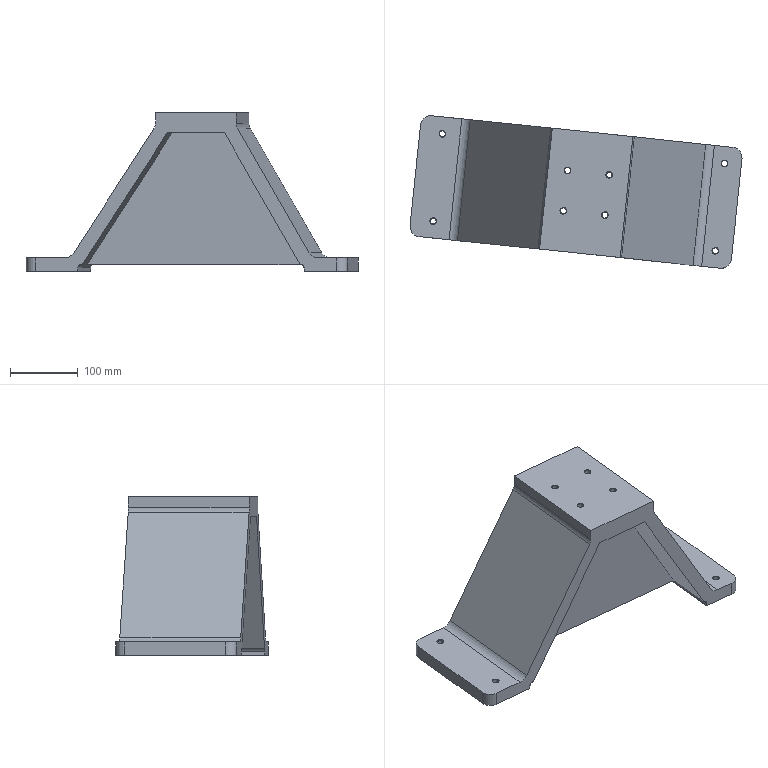Component | NX | BRACKET | 1 solid | 58 faces | volume 4355076 mm3 | plane 24 | cylinder 18 | cone 16 | commonest cylinder face diameters 8.5 x8 30 x8 10 x2